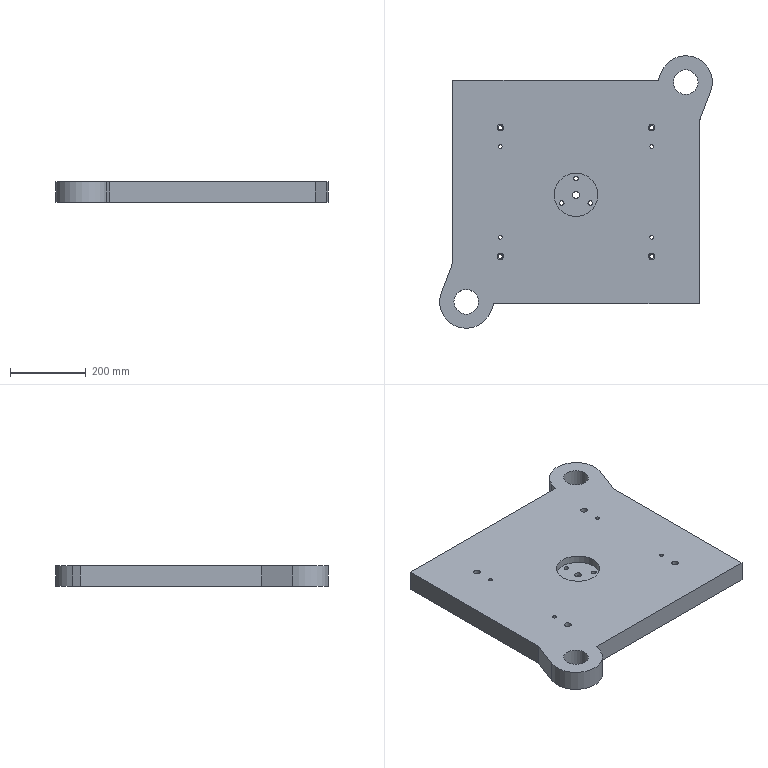Component | NX | UPPER_DIE_BASE | 1 solid | 50 faces | volume 19918548 mm3 | cylinder 25 | plane 19 | cone 6 | commonest cylinder face diameters 11 x4 10 x4 17 x4 11.701 x3 40 x3 140 x2 65 x2 18 x1